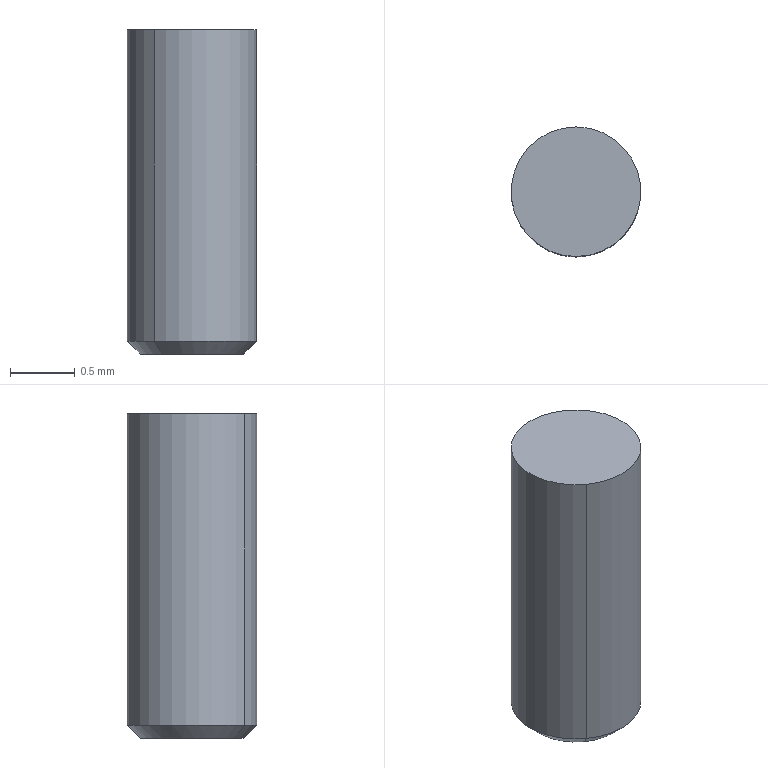Component | SolidWorks | Part5^Assembly1-4 | 1 solid | 6 faces | box 1 x 1 x 2.5 mm | volume 2 mm3 | cone 2 | cylinder 2 | plane 2 | commonest cylinder face diameters 1 x2
STEP:
#1=COLOUR_RGB('',0.7922,0.8196,0.9333);
#2=FILL_AREA_STYLE_COLOUR('',#1);
#3=FILL_AREA_STYLE('',(#2));
#4=SURFACE_STYLE_FILL_AREA(#3);
#5=SURFACE_SIDE_STYLE('',(#4));
#6=SURFACE_STYLE_USAGE(.BOTH.,#5);
#7=PRESENTATION_STYLE_ASSIGNMENT((#6));
#8=CARTESIAN_POINT('',(-0.5073,-0.08272,-0.2953));
#9=VERTEX_POINT('',#8);
#10=CARTESIAN_POINT('',(-0.489,-0.05715,-0.2953));
#11=VERTEX_POINT('',#10);
#12=CARTESIAN_POINT('',(-0.4982,-0.06993,-0.2953));
#13=DIRECTION('',(0.,0.,-1.));
#14=DIRECTION('',(-0.5836,-0.812,-0.));
#15=AXIS2_PLACEMENT_3D('',#12,#13,#14);
#16=CIRCLE('',#15,0.01575);
#17=EDGE_CURVE('',#9,#11,#16,.T.);
#18=ORIENTED_EDGE('',*,*,#17,.F.);
#19=CARTESIAN_POINT('',(-0.5096,-0.08592,-0.2913));
#20=VERTEX_POINT('',#19);
#21=CARTESIAN_POINT('',(-0.5073,-0.08272,-0.2953));
#22=DIRECTION('',(-0.4127,-0.5742,0.7071));
#23=VECTOR('',#22,39.37);
#24=LINE('',#21,#23);
#25=EDGE_CURVE('',#9,#20,#24,.T.);
#26=ORIENTED_EDGE('',*,*,#25,.T.);
#27=CARTESIAN_POINT('',(-0.4867,-0.05395,-0.2913));
#28=VERTEX_POINT('',#27);
#29=CARTESIAN_POINT('',(-0.4982,-0.06993,-0.2913));
#30=DIRECTION('',(-0.,-0.,1.));
#31=DIRECTION('',(-0.5836,-0.812,-0.));
#32=AXIS2_PLACEMENT_3D('',#29,#30,#31);
#33=CIRCLE('',#32,0.01969);
#34=EDGE_CURVE('',#28,#20,#33,.T.);
#35=ORIENTED_EDGE('',*,*,#34,.F.);
#36=CARTESIAN_POINT('',(-0.489,-0.05715,-0.2953));
#37=DIRECTION('',(0.4127,0.5742,0.7071));
#38=VECTOR('',#37,39.37);
#39=LINE('',#36,#38);
#40=EDGE_CURVE('',#11,#28,#39,.T.);
#41=ORIENTED_EDGE('',*,*,#40,.F.);
#42=EDGE_LOOP('',(#18,#26,#35,#41));
#43=FACE_OUTER_BOUND('',#42,.T.);
#44=CARTESIAN_POINT('',(-0.4982,-0.06993,-0.2953));
#45=DIRECTION('',(-0.,-0.,1.));
#46=DIRECTION('',(0.5836,0.812,0.));
#47=AXIS2_PLACEMENT_3D('',#44,#45,#46);
#48=CONICAL_SURFACE('',#47,0.01575,0.7854);
#49=ADVANCED_FACE('',(#43),#48,.T.);
#50=ORIENTED_EDGE('',*,*,#34,.T.);
#51=CARTESIAN_POINT('',(-0.5096,-0.08592,-0.1969));
#52=VERTEX_POINT('',#51);
#53=CARTESIAN_POINT('',(-0.5096,-0.08592,-0.2953));
#54=DIRECTION('',(-0.,-0.,1.));
#55=VECTOR('',#54,39.37);
#56=LINE('',#53,#55);
#57=EDGE_CURVE('',#20,#52,#56,.T.);
#58=ORIENTED_EDGE('',*,*,#57,.T.);
#59=CARTESIAN_POINT('',(-0.4867,-0.05395,-0.1969));
#60=VERTEX_POINT('',#59);
#61=CARTESIAN_POINT('',(-0.4982,-0.06993,-0.1969));
#62=DIRECTION('',(0.,0.,-1.));
#63=DIRECTION('',(-0.5836,-0.812,-0.));
#64=AXIS2_PLACEMENT_3D('',#61,#62,#63);
#65=CIRCLE('',#64,0.01969);
#66=EDGE_CURVE('',#52,#60,#65,.T.);
#67=ORIENTED_EDGE('',*,*,#66,.T.);
#68=CARTESIAN_POINT('',(-0.4867,-0.05395,-0.2953));
#69=DIRECTION('',(-0.,-0.,1.));
#70=VECTOR('',#69,39.37);
#71=LINE('',#68,#70);
#72=EDGE_CURVE('',#28,#60,#71,.T.);
#73=ORIENTED_EDGE('',*,*,#72,.F.);
#74=EDGE_LOOP('',(#50,#58,#67,#73));
#75=FACE_OUTER_BOUND('',#74,.T.);
#76=CARTESIAN_POINT('',(-0.4982,-0.06993,-0.2953));
#77=DIRECTION('',(-0.,-0.,1.));
#78=DIRECTION('',(0.5836,0.812,0.));
#79=AXIS2_PLACEMENT_3D('',#76,#77,#78);
#80=CYLINDRICAL_SURFACE('',#79,0.01969);
#81=ADVANCED_FACE('',(#75),#80,.T.);
#82=ORIENTED_EDGE('',*,*,#57,.F.);
#83=CARTESIAN_POINT('',(-0.4982,-0.06993,-0.2913));
#84=DIRECTION('',(-0.,-0.,1.));
#85=DIRECTION('',(-0.5836,-0.812,-0.));
#86=AXIS2_PLACEMENT_3D('',#83,#84,#85);
#87=CIRCLE('',#86,0.01969);
#88=EDGE_CURVE('',#20,#28,#87,.T.);
#89=ORIENTED_EDGE('',*,*,#88,.T.);
#90=ORIENTED_EDGE('',*,*,#72,.T.);
#91=CARTESIAN_POINT('',(-0.4982,-0.06993,-0.1969));
#92=DIRECTION('',(0.,0.,-1.));
#93=DIRECTION('',(-0.5836,-0.812,-0.));
#94=AXIS2_PLACEMENT_3D('',#91,#92,#93);
#95=CIRCLE('',#94,0.01969);
#96=EDGE_CURVE('',#60,#52,#95,.T.);
#97=ORIENTED_EDGE('',*,*,#96,.T.);
#98=EDGE_LOOP('',(#82,#89,#90,#97));
#99=FACE_OUTER_BOUND('',#98,.T.);
#100=CARTESIAN_POINT('',(-0.4982,-0.06993,-0.2953));
#101=DIRECTION('',(-0.,-0.,1.));
#102=DIRECTION('',(0.5836,0.812,0.));
#103=AXIS2_PLACEMENT_3D('',#100,#101,#102);
#104=CYLINDRICAL_SURFACE('',#103,0.01969);
#105=ADVANCED_FACE('',(#99),#104,.T.);
#106=CARTESIAN_POINT('',(-0.4982,-0.06993,-0.2953));
#107=DIRECTION('',(0.,0.,-1.));
#108=DIRECTION('',(-0.5836,-0.812,-0.));
#109=AXIS2_PLACEMENT_3D('',#106,#107,#108);
#110=CIRCLE('',#109,0.01575);
#111=EDGE_CURVE('',#11,#9,#110,.T.);
#112=ORIENTED_EDGE('',*,*,#111,.T.);
#113=ORIENTED_EDGE('',*,*,#17,.T.);
#114=EDGE_LOOP('',(#112,#113));
#115=FACE_OUTER_BOUND('',#114,.T.);
#116=CARTESIAN_POINT('',(-0.4982,-0.06993,-0.2953));
#117=DIRECTION('',(0.,0.,-1.));
#118=DIRECTION('',(-0.5836,-0.812,-0.));
#119=AXIS2_PLACEMENT_3D('',#116,#117,#118);
#120=PLANE('',#119);
#121=ADVANCED_FACE('',(#115),#120,.T.);
#122=ORIENTED_EDGE('',*,*,#96,.F.);
#123=ORIENTED_EDGE('',*,*,#66,.F.);
#124=EDGE_LOOP('',(#122,#123));
#125=FACE_OUTER_BOUND('',#124,.T.);
#126=CARTESIAN_POINT('',(-0.4982,-0.06993,-0.1969));
#127=DIRECTION('',(0.,0.,-1.));
#128=DIRECTION('',(-0.5836,-0.812,-0.));
#129=AXIS2_PLACEMENT_3D('',#126,#127,#128);
#130=PLANE('',#129);
#131=ADVANCED_FACE('',(#125),#130,.F.);
#132=ORIENTED_EDGE('',*,*,#25,.F.);
#133=ORIENTED_EDGE('',*,*,#111,.F.);
#134=ORIENTED_EDGE('',*,*,#40,.T.);
#135=ORIENTED_EDGE('',*,*,#88,.F.);
#136=EDGE_LOOP('',(#132,#133,#134,#135));
#137=FACE_OUTER_BOUND('',#136,.T.);
#138=CARTESIAN_POINT('',(-0.4982,-0.06993,-0.2953));
#139=DIRECTION('',(-0.,-0.,1.));
#140=DIRECTION('',(0.5836,0.812,0.));
#141=AXIS2_PLACEMENT_3D('',#138,#139,#140);
#142=CONICAL_SURFACE('',#141,0.01575,0.7854);
#143=ADVANCED_FACE('',(#137),#142,.T.);
#144=CLOSED_SHELL('',(#49,#81,#105,#121,#131,#143));
#145=MANIFOLD_SOLID_BREP('',#144);
#146=STYLED_ITEM('',(#7),#145);
#147=PRESENTATION_LAYER_ASSIGNMENT('','',(#146));
#148=CARTESIAN_POINT('',(0.,0.,0.));
#149=DIRECTION('',(0.,0.,1.));
#150=DIRECTION('',(1.,0.,0.));
#151=AXIS2_PLACEMENT_3D('',#148,#149,#150);
#152=(LENGTH_UNIT()NAMED_UNIT(*)SI_UNIT($,.METRE.));
#153=LENGTH_MEASURE_WITH_UNIT(LENGTH_MEASURE(0.0254),#152);
#154=DIMENSIONAL_EXPONENTS(1.,0.,0.,0.,0.,0.,0.);
#155=(CONVERSION_BASED_UNIT('',#153)LENGTH_UNIT()NAMED_UNIT(#154));
#156=UNCERTAINTY_MEASURE_WITH_UNIT(LENGTH_MEASURE(0.00001),#155,'','');
#157=(NAMED_UNIT(*)PLANE_ANGLE_UNIT()SI_UNIT($,.RADIAN.));
#158=(NAMED_UNIT(*)SI_UNIT($,.STERADIAN.)SOLID_ANGLE_UNIT());
#159=(GEOMETRIC_REPRESENTATION_CONTEXT(3)GLOBAL_UNCERTAINTY_ASSIGNED_CONTEXT((#156))GLOBAL_UNIT_ASSIGNED_CONTEXT((#155,#157,#158))REPRESENTATION_CONTEXT('',''));
#160=ADVANCED_BREP_SHAPE_REPRESENTATION('',(#145,#151),#159);
#161=(LENGTH_UNIT()NAMED_UNIT(*)SI_UNIT($,.METRE.));
#162=LENGTH_MEASURE_WITH_UNIT(LENGTH_MEASURE(0.0254),#161);
#163=DIMENSIONAL_EXPONENTS(1.,0.,0.,0.,0.,0.,0.);
#164=(CONVERSION_BASED_UNIT('',#162)LENGTH_UNIT()NAMED_UNIT(#163));
#165=UNCERTAINTY_MEASURE_WITH_UNIT(LENGTH_MEASURE(0.00001),#164,'','');
#166=(NAMED_UNIT(*)PLANE_ANGLE_UNIT()SI_UNIT($,.RADIAN.));
#167=(NAMED_UNIT(*)SI_UNIT($,.STERADIAN.)SOLID_ANGLE_UNIT());
#168=(GEOMETRIC_REPRESENTATION_CONTEXT(3)GLOBAL_UNCERTAINTY_ASSIGNED_CONTEXT((#165))GLOBAL_UNIT_ASSIGNED_CONTEXT((#164,#166,#167))REPRESENTATION_CONTEXT('',''));
#169=MECHANICAL_DESIGN_GEOMETRIC_PRESENTATION_REPRESENTATION('',(#146),#168);